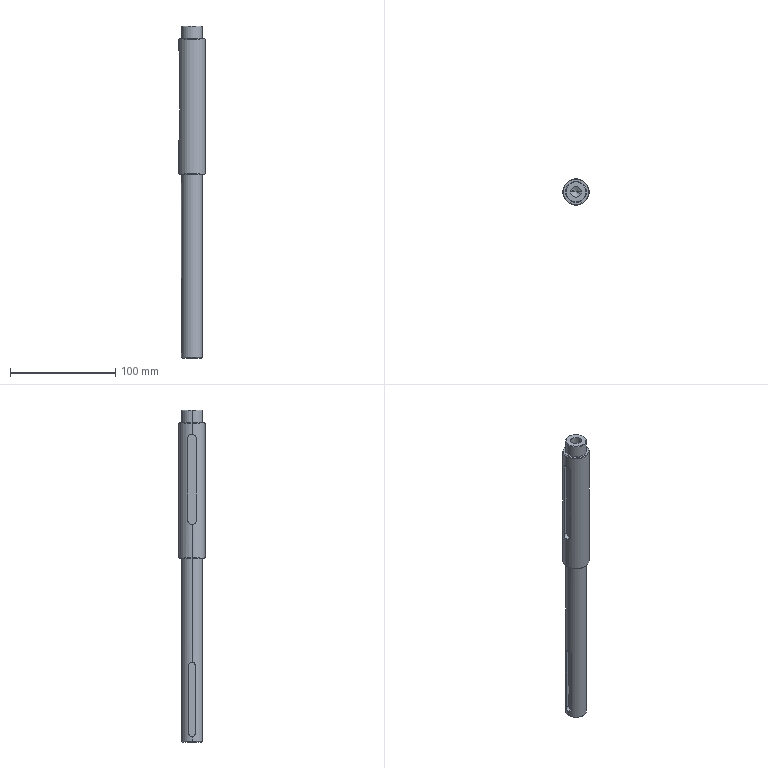Component | SolidWorks | TractionDriveWheelAssembly-1_TractionDriveAxis-1 | 1 solid | 34 faces | box 25 x 25 x 316 mm | volume 116078 mm3 | cylinder 14 | cone 10 | plane 10 | commonest cylinder face diameters 20 x4 6 x3 8 x3 10 x2 25 x2
STEP:
#1=CARTESIAN_POINT('',(-11.988,-1.571,24.075));
#2=VERTEX_POINT('',#1);
#3=CARTESIAN_POINT('',(-11.595,-1.571,24.075));
#4=VERTEX_POINT('',#3);
#5=CARTESIAN_POINT('',(-11.792,-1.571,24.075));
#6=DIRECTION('',(-0.,-0.,1.));
#7=DIRECTION('',(1.,0.,0.));
#8=AXIS2_PLACEMENT_3D('',#5,#6,#7);
#9=CIRCLE('',#8,0.1969);
#10=EDGE_CURVE('',#2,#4,#9,.T.);
#11=ORIENTED_EDGE('',*,*,#10,.F.);
#12=CARTESIAN_POINT('',(-11.988,-1.571,25.039));
#13=VERTEX_POINT('',#12);
#14=CARTESIAN_POINT('',(-11.988,-1.571,25.039));
#15=DIRECTION('',(-0.,-0.,1.));
#16=VECTOR('',#15,39.37);
#17=LINE('',#14,#16);
#18=EDGE_CURVE('',#2,#13,#17,.T.);
#19=ORIENTED_EDGE('',*,*,#18,.T.);
#20=CARTESIAN_POINT('',(-11.595,-1.571,25.039));
#21=VERTEX_POINT('',#20);
#22=CARTESIAN_POINT('',(-11.792,-1.571,25.039));
#23=DIRECTION('',(-0.,-0.,1.));
#24=DIRECTION('',(1.,0.,0.));
#25=AXIS2_PLACEMENT_3D('',#22,#23,#24);
#26=CIRCLE('',#25,0.1969);
#27=EDGE_CURVE('',#13,#21,#26,.T.);
#28=ORIENTED_EDGE('',*,*,#27,.T.);
#29=CARTESIAN_POINT('',(-11.595,-1.571,25.039));
#30=DIRECTION('',(-0.,-0.,1.));
#31=VECTOR('',#30,39.37);
#32=LINE('',#29,#31);
#33=EDGE_CURVE('',#4,#21,#32,.T.);
#34=ORIENTED_EDGE('',*,*,#33,.F.);
#35=EDGE_LOOP('',(#11,#19,#28,#34));
#36=FACE_OUTER_BOUND('',#35,.T.);
#37=CARTESIAN_POINT('',(-11.792,-1.571,25.039));
#38=DIRECTION('',(-0.,-0.,1.));
#39=DIRECTION('',(1.,0.,0.));
#40=AXIS2_PLACEMENT_3D('',#37,#38,#39);
#41=CYLINDRICAL_SURFACE('',#40,0.1969);
#42=ADVANCED_FACE('',(#36),#41,.F.);
#43=CARTESIAN_POINT('',(-11.792,-1.571,23.957));
#44=VERTEX_POINT('',#43);
#45=CARTESIAN_POINT('',(-11.595,-1.571,24.075));
#46=DIRECTION('',(0.8572,0.,0.515));
#47=VECTOR('',#46,39.37);
#48=LINE('',#45,#47);
#49=EDGE_CURVE('',#44,#4,#48,.T.);
#50=ORIENTED_EDGE('',*,*,#49,.F.);
#51=CARTESIAN_POINT('',(-11.988,-1.571,24.075));
#52=DIRECTION('',(-0.8572,-0.,0.515));
#53=VECTOR('',#52,39.37);
#54=LINE('',#51,#53);
#55=EDGE_CURVE('',#44,#2,#54,.T.);
#56=ORIENTED_EDGE('',*,*,#55,.T.);
#57=ORIENTED_EDGE('',*,*,#10,.T.);
#58=EDGE_LOOP('',(#50,#56,#57));
#59=FACE_OUTER_BOUND('',#58,.T.);
#60=CARTESIAN_POINT('',(-11.792,-1.571,24.075));
#61=DIRECTION('',(-0.,-0.,1.));
#62=DIRECTION('',(1.,0.,0.));
#63=AXIS2_PLACEMENT_3D('',#60,#61,#62);
#64=CONICAL_SURFACE('',#63,0.1969,1.03);
#65=ADVANCED_FACE('',(#59),#64,.F.);
#66=CARTESIAN_POINT('',(-12.185,-1.571,12.795));
#67=VERTEX_POINT('',#66);
#68=CARTESIAN_POINT('',(-12.167,-1.453,12.913));
#69=VERTEX_POINT('',#68);
#70=CARTESIAN_POINT('',(-12.185,-1.571,12.795));
#71=CARTESIAN_POINT('',(-12.185,-1.564,12.795));
#72=CARTESIAN_POINT('',(-12.185,-1.556,12.796));
#73=CARTESIAN_POINT('',(-12.184,-1.541,12.799));
#74=CARTESIAN_POINT('',(-12.184,-1.533,12.801));
#75=CARTESIAN_POINT('',(-12.182,-1.519,12.807));
#76=CARTESIAN_POINT('',(-12.181,-1.512,12.811));
#77=CARTESIAN_POINT('',(-12.179,-1.499,12.82));
#78=CARTESIAN_POINT('',(-12.178,-1.493,12.824));
#79=CARTESIAN_POINT('',(-12.175,-1.482,12.835));
#80=CARTESIAN_POINT('',(-12.174,-1.477,12.841));
#81=CARTESIAN_POINT('',(-12.172,-1.469,12.854));
#82=CARTESIAN_POINT('',(-12.171,-1.465,12.861));
#83=CARTESIAN_POINT('',(-12.169,-1.459,12.875));
#84=CARTESIAN_POINT('',(-12.168,-1.457,12.882));
#85=CARTESIAN_POINT('',(-12.167,-1.454,12.898));
#86=CARTESIAN_POINT('',(-12.167,-1.453,12.906));
#87=CARTESIAN_POINT('',(-12.167,-1.453,12.913));
#88=B_SPLINE_CURVE_WITH_KNOTS('',3,(#70,#71,#72,#73,#74,#75,#76,#77,#78,#79,#80,#81,#82,#83,#84,#85,#86,#87),.UNSPECIFIED.,.F.,.F.,(4,2,2,2,2,2,2,2,4),(0.004718,0.005307,0.005896,0.006485,0.007074,0.007663,0.008252,0.008842,0.009431),.UNSPECIFIED.);
#89=EDGE_CURVE('',#67,#69,#88,.T.);
#90=ORIENTED_EDGE('',*,*,#89,.F.);
#91=CARTESIAN_POINT('',(-12.048,-1.571,12.795));
#92=VERTEX_POINT('',#91);
#93=CARTESIAN_POINT('',(-12.284,-1.571,12.795));
#94=DIRECTION('',(1.,0.,0.));
#95=VECTOR('',#94,39.37);
#96=LINE('',#93,#95);
#97=EDGE_CURVE('',#67,#92,#96,.T.);
#98=ORIENTED_EDGE('',*,*,#97,.T.);
#99=CARTESIAN_POINT('',(-12.048,-1.453,12.913));
#100=VERTEX_POINT('',#99);
#101=CARTESIAN_POINT('',(-12.048,-1.571,12.913));
#102=DIRECTION('',(1.,0.,0.));
#103=DIRECTION('',(0.,0.,-1.));
#104=AXIS2_PLACEMENT_3D('',#101,#102,#103);
#105=CIRCLE('',#104,0.1181);
#106=EDGE_CURVE('',#92,#100,#105,.T.);
#107=ORIENTED_EDGE('',*,*,#106,.T.);
#108=CARTESIAN_POINT('',(-12.284,-1.453,12.913));
#109=DIRECTION('',(1.,0.,0.));
#110=VECTOR('',#109,39.37);
#111=LINE('',#108,#110);
#112=EDGE_CURVE('',#69,#100,#111,.T.);
#113=ORIENTED_EDGE('',*,*,#112,.F.);
#114=EDGE_LOOP('',(#90,#98,#107,#113));
#115=FACE_OUTER_BOUND('',#114,.T.);
#116=CARTESIAN_POINT('',(-12.284,-1.571,12.913));
#117=DIRECTION('',(1.,0.,0.));
#118=DIRECTION('',(0.,0.,-1.));
#119=AXIS2_PLACEMENT_3D('',#116,#117,#118);
#120=CYLINDRICAL_SURFACE('',#119,0.1181);
#121=ADVANCED_FACE('',(#115),#120,.F.);
#122=CARTESIAN_POINT('',(-11.398,-1.571,12.618));
#123=VERTEX_POINT('',#122);
#124=CARTESIAN_POINT('',(-12.185,-1.571,12.618));
#125=VERTEX_POINT('',#124);
#126=CARTESIAN_POINT('',(-11.792,-1.571,12.618));
#127=DIRECTION('',(-0.,-0.,1.));
#128=DIRECTION('',(1.,0.,0.));
#129=AXIS2_PLACEMENT_3D('',#126,#127,#128);
#130=CIRCLE('',#129,0.3937);
#131=EDGE_CURVE('',#123,#125,#130,.T.);
#132=ORIENTED_EDGE('',*,*,#131,.T.);
#133=CARTESIAN_POINT('',(-12.185,-1.571,38.002));
#134=DIRECTION('',(-0.,-0.,1.));
#135=VECTOR('',#134,39.37);
#136=LINE('',#133,#135);
#137=EDGE_CURVE('',#125,#67,#136,.T.);
#138=ORIENTED_EDGE('',*,*,#137,.T.);
#139=ORIENTED_EDGE('',*,*,#89,.T.);
#140=CARTESIAN_POINT('',(-12.167,-1.453,15.472));
#141=VERTEX_POINT('',#140);
#142=CARTESIAN_POINT('',(-12.167,-1.453,38.002));
#143=DIRECTION('',(-0.,-0.,1.));
#144=VECTOR('',#143,39.37);
#145=LINE('',#142,#144);
#146=EDGE_CURVE('',#69,#141,#145,.T.);
#147=ORIENTED_EDGE('',*,*,#146,.T.);
#148=CARTESIAN_POINT('',(-12.185,-1.571,15.591));
#149=VERTEX_POINT('',#148);
#150=CARTESIAN_POINT('',(-12.167,-1.453,15.472));
#151=CARTESIAN_POINT('',(-12.167,-1.453,15.48));
#152=CARTESIAN_POINT('',(-12.167,-1.454,15.488));
#153=CARTESIAN_POINT('',(-12.168,-1.457,15.503));
#154=CARTESIAN_POINT('',(-12.169,-1.459,15.511));
#155=CARTESIAN_POINT('',(-12.171,-1.465,15.525));
#156=CARTESIAN_POINT('',(-12.172,-1.469,15.532));
#157=CARTESIAN_POINT('',(-12.174,-1.477,15.545));
#158=CARTESIAN_POINT('',(-12.175,-1.482,15.551));
#159=CARTESIAN_POINT('',(-12.179,-1.499,15.567));
#160=CARTESIAN_POINT('',(-12.181,-1.512,15.576));
#161=CARTESIAN_POINT('',(-12.184,-1.533,15.584));
#162=CARTESIAN_POINT('',(-12.184,-1.541,15.587));
#163=CARTESIAN_POINT('',(-12.185,-1.556,15.59));
#164=CARTESIAN_POINT('',(-12.185,-1.564,15.591));
#165=CARTESIAN_POINT('',(-12.185,-1.571,15.591));
#166=B_SPLINE_CURVE_WITH_KNOTS('',3,(#150,#151,#152,#153,#154,#155,#156,#157,#158,#159,#160,#161,#162,#163,#164,#165),.UNSPECIFIED.,.F.,.F.,(4,2,2,2,2,2,2,4),(0.,0.0005898,0.00118,0.001769,0.002359,0.003539,0.004128,0.004718),.UNSPECIFIED.);
#167=EDGE_CURVE('',#141,#149,#166,.T.);
#168=ORIENTED_EDGE('',*,*,#167,.T.);
#169=CARTESIAN_POINT('',(-12.185,-1.571,19.488));
#170=VERTEX_POINT('',#169);
#171=CARTESIAN_POINT('',(-12.185,-1.571,38.002));
#172=DIRECTION('',(-0.,-0.,1.));
#173=VECTOR('',#172,39.37);
#174=LINE('',#171,#173);
#175=EDGE_CURVE('',#149,#170,#174,.T.);
#176=ORIENTED_EDGE('',*,*,#175,.T.);
#177=CARTESIAN_POINT('',(-11.398,-1.571,19.488));
#178=VERTEX_POINT('',#177);
#179=CARTESIAN_POINT('',(-11.792,-1.571,19.488));
#180=DIRECTION('',(-0.,-0.,1.));
#181=DIRECTION('',(1.,0.,0.));
#182=AXIS2_PLACEMENT_3D('',#179,#180,#181);
#183=CIRCLE('',#182,0.3937);
#184=EDGE_CURVE('',#178,#170,#183,.T.);
#185=ORIENTED_EDGE('',*,*,#184,.F.);
#186=CARTESIAN_POINT('',(-11.398,-1.571,38.002));
#187=DIRECTION('',(-0.,-0.,1.));
#188=VECTOR('',#187,39.37);
#189=LINE('',#186,#188);
#190=EDGE_CURVE('',#123,#178,#189,.T.);
#191=ORIENTED_EDGE('',*,*,#190,.F.);
#192=EDGE_LOOP('',(#132,#138,#139,#147,#168,#176,#185,#191));
#193=FACE_OUTER_BOUND('',#192,.T.);
#194=CARTESIAN_POINT('',(-11.792,-1.571,38.002));
#195=DIRECTION('',(-0.,-0.,1.));
#196=DIRECTION('',(1.,0.,0.));
#197=AXIS2_PLACEMENT_3D('',#194,#195,#196);
#198=CYLINDRICAL_SURFACE('',#197,0.3937);
#199=ADVANCED_FACE('',(#193),#198,.T.);
#200=CARTESIAN_POINT('',(-12.166,-1.571,12.598));
#201=VERTEX_POINT('',#200);
#202=CARTESIAN_POINT('',(-11.418,-1.571,12.598));
#203=VERTEX_POINT('',#202);
#204=CARTESIAN_POINT('',(-11.792,-1.571,12.598));
#205=DIRECTION('',(0.,0.,-1.));
#206=DIRECTION('',(1.,0.,0.));
#207=AXIS2_PLACEMENT_3D('',#204,#205,#206);
#208=CIRCLE('',#207,0.374);
#209=EDGE_CURVE('',#201,#203,#208,.T.);
#210=ORIENTED_EDGE('',*,*,#209,.F.);
#211=CARTESIAN_POINT('',(-12.185,-1.571,12.618));
#212=DIRECTION('',(-0.7071,-0.,0.7071));
#213=VECTOR('',#212,39.37);
#214=LINE('',#211,#213);
#215=EDGE_CURVE('',#201,#125,#214,.T.);
#216=ORIENTED_EDGE('',*,*,#215,.T.);
#217=ORIENTED_EDGE('',*,*,#131,.F.);
#218=CARTESIAN_POINT('',(-11.398,-1.571,12.618));
#219=DIRECTION('',(0.7071,0.,0.7071));
#220=VECTOR('',#219,39.37);
#221=LINE('',#218,#220);
#222=EDGE_CURVE('',#203,#123,#221,.T.);
#223=ORIENTED_EDGE('',*,*,#222,.F.);
#224=EDGE_LOOP('',(#210,#216,#217,#223));
#225=FACE_OUTER_BOUND('',#224,.T.);
#226=CARTESIAN_POINT('',(-11.792,-1.571,12.618));
#227=DIRECTION('',(-0.,-0.,1.));
#228=DIRECTION('',(1.,0.,0.));
#229=AXIS2_PLACEMENT_3D('',#226,#227,#228);
#230=CONICAL_SURFACE('',#229,0.3937,0.7854);
#231=ADVANCED_FACE('',(#225),#230,.T.);
#232=CARTESIAN_POINT('',(-11.319,-1.571,24.567));
#233=VERTEX_POINT('',#232);
#234=CARTESIAN_POINT('',(-12.264,-1.571,24.567));
#235=VERTEX_POINT('',#234);
#236=CARTESIAN_POINT('',(-11.792,-1.571,24.567));
#237=DIRECTION('',(-0.,-0.,1.));
#238=DIRECTION('',(-1.,-0.,0.));
#239=AXIS2_PLACEMENT_3D('',#236,#237,#238);
#240=CIRCLE('',#239,0.4724);
#241=EDGE_CURVE('',#233,#235,#240,.T.);
#242=ORIENTED_EDGE('',*,*,#241,.F.);
#243=CARTESIAN_POINT('',(-11.299,-1.571,24.547));
#244=VERTEX_POINT('',#243);
#245=CARTESIAN_POINT('',(-11.319,-1.571,24.567));
#246=DIRECTION('',(0.7071,0.,-0.7071));
#247=VECTOR('',#246,39.37);
#248=LINE('',#245,#247);
#249=EDGE_CURVE('',#233,#244,#248,.T.);
#250=ORIENTED_EDGE('',*,*,#249,.T.);
#251=CARTESIAN_POINT('',(-12.284,-1.571,24.547));
#252=VERTEX_POINT('',#251);
#253=CARTESIAN_POINT('',(-11.792,-1.571,24.547));
#254=DIRECTION('',(0.,0.,-1.));
#255=DIRECTION('',(-1.,-0.,0.));
#256=AXIS2_PLACEMENT_3D('',#253,#254,#255);
#257=CIRCLE('',#256,0.4921);
#258=EDGE_CURVE('',#252,#244,#257,.T.);
#259=ORIENTED_EDGE('',*,*,#258,.F.);
#260=CARTESIAN_POINT('',(-12.264,-1.571,24.567));
#261=DIRECTION('',(-0.7071,-0.,-0.7071));
#262=VECTOR('',#261,39.37);
#263=LINE('',#260,#262);
#264=EDGE_CURVE('',#235,#252,#263,.T.);
#265=ORIENTED_EDGE('',*,*,#264,.F.);
#266=EDGE_LOOP('',(#242,#250,#259,#265));
#267=FACE_OUTER_BOUND('',#266,.T.);
#268=CARTESIAN_POINT('',(-11.792,-1.571,24.567));
#269=DIRECTION('',(0.,0.,-1.));
#270=DIRECTION('',(-1.,-0.,0.));
#271=AXIS2_PLACEMENT_3D('',#268,#269,#270);
#272=CONICAL_SURFACE('',#271,0.4724,0.7854);
#273=ADVANCED_FACE('',(#267),#272,.T.);
#274=CARTESIAN_POINT('',(-11.398,-1.571,24.567));
#275=VERTEX_POINT('',#274);
#276=CARTESIAN_POINT('',(-12.185,-1.571,24.567));
#277=VERTEX_POINT('',#276);
#278=CARTESIAN_POINT('',(-11.792,-1.571,24.567));
#279=DIRECTION('',(-0.,-0.,1.));
#280=DIRECTION('',(1.,0.,0.));
#281=AXIS2_PLACEMENT_3D('',#278,#279,#280);
#282=CIRCLE('',#281,0.3937);
#283=EDGE_CURVE('',#275,#277,#282,.T.);
#284=ORIENTED_EDGE('',*,*,#283,.T.);
#285=CARTESIAN_POINT('',(-12.185,-1.571,25.02));
#286=VERTEX_POINT('',#285);
#287=CARTESIAN_POINT('',(-12.185,-1.571,38.002));
#288=DIRECTION('',(-0.,-0.,1.));
#289=VECTOR('',#288,39.37);
#290=LINE('',#287,#289);
#291=EDGE_CURVE('',#277,#286,#290,.T.);
#292=ORIENTED_EDGE('',*,*,#291,.T.);
#293=CARTESIAN_POINT('',(-11.398,-1.571,25.02));
#294=VERTEX_POINT('',#293);
#295=CARTESIAN_POINT('',(-11.792,-1.571,25.02));
#296=DIRECTION('',(0.,0.,-1.));
#297=DIRECTION('',(-1.,-0.,0.));
#298=AXIS2_PLACEMENT_3D('',#295,#296,#297);
#299=CIRCLE('',#298,0.3937);
#300=EDGE_CURVE('',#286,#294,#299,.T.);
#301=ORIENTED_EDGE('',*,*,#300,.T.);
#302=CARTESIAN_POINT('',(-11.398,-1.571,38.002));
#303=DIRECTION('',(-0.,-0.,1.));
#304=VECTOR('',#303,39.37);
#305=LINE('',#302,#304);
#306=EDGE_CURVE('',#275,#294,#305,.T.);
#307=ORIENTED_EDGE('',*,*,#306,.F.);
#308=EDGE_LOOP('',(#284,#292,#301,#307));
#309=FACE_OUTER_BOUND('',#308,.T.);
#310=CARTESIAN_POINT('',(-11.792,-1.571,38.002));
#311=DIRECTION('',(-0.,-0.,1.));
#312=DIRECTION('',(1.,0.,0.));
#313=AXIS2_PLACEMENT_3D('',#310,#311,#312);
#314=CYLINDRICAL_SURFACE('',#313,0.3937);
#315=ADVANCED_FACE('',(#309),#314,.T.);
#316=CARTESIAN_POINT('',(-11.418,-1.571,25.039));
#317=VERTEX_POINT('',#316);
#318=CARTESIAN_POINT('',(-12.166,-1.571,25.039));
#319=VERTEX_POINT('',#318);
#320=CARTESIAN_POINT('',(-11.792,-1.571,25.039));
#321=DIRECTION('',(-0.,-0.,1.));
#322=DIRECTION('',(-1.,-0.,0.));
#323=AXIS2_PLACEMENT_3D('',#320,#321,#322);
#324=CIRCLE('',#323,0.374);
#325=EDGE_CURVE('',#317,#319,#324,.T.);
#326=ORIENTED_EDGE('',*,*,#325,.F.);
#327=CARTESIAN_POINT('',(-11.418,-1.571,25.039));
#328=DIRECTION('',(0.7071,0.,-0.7071));
#329=VECTOR('',#328,39.37);
#330=LINE('',#327,#329);
#331=EDGE_CURVE('',#317,#294,#330,.T.);
#332=ORIENTED_EDGE('',*,*,#331,.T.);
#333=ORIENTED_EDGE('',*,*,#300,.F.);
#334=CARTESIAN_POINT('',(-12.166,-1.571,25.039));
#335=DIRECTION('',(-0.7071,-0.,-0.7071));
#336=VECTOR('',#335,39.37);
#337=LINE('',#334,#336);
#338=EDGE_CURVE('',#319,#286,#337,.T.);
#339=ORIENTED_EDGE('',*,*,#338,.F.);
#340=EDGE_LOOP('',(#326,#332,#333,#339));
#341=FACE_OUTER_BOUND('',#340,.T.);
#342=CARTESIAN_POINT('',(-11.792,-1.571,25.039));
#343=DIRECTION('',(0.,0.,-1.));
#344=DIRECTION('',(-1.,-0.,0.));
#345=AXIS2_PLACEMENT_3D('',#342,#343,#344);
#346=CONICAL_SURFACE('',#345,0.374,0.7854);
#347=ADVANCED_FACE('',(#341),#346,.T.);
#348=CARTESIAN_POINT('',(-12.284,-1.571,20.748));
#349=VERTEX_POINT('',#348);
#350=CARTESIAN_POINT('',(-12.258,-1.414,20.906));
#351=VERTEX_POINT('',#350);
#352=CARTESIAN_POINT('',(-12.284,-1.571,20.748));
#353=CARTESIAN_POINT('',(-12.284,-1.561,20.748));
#354=CARTESIAN_POINT('',(-12.283,-1.55,20.749));
#355=CARTESIAN_POINT('',(-12.282,-1.53,20.753));
#356=CARTESIAN_POINT('',(-12.281,-1.52,20.756));
#357=CARTESIAN_POINT('',(-12.279,-1.501,20.764));
#358=CARTESIAN_POINT('',(-12.277,-1.492,20.769));
#359=CARTESIAN_POINT('',(-12.274,-1.475,20.78));
#360=CARTESIAN_POINT('',(-12.273,-1.467,20.787));
#361=CARTESIAN_POINT('',(-12.269,-1.453,20.801));
#362=CARTESIAN_POINT('',(-12.268,-1.446,20.809));
#363=CARTESIAN_POINT('',(-12.264,-1.435,20.826));
#364=CARTESIAN_POINT('',(-12.263,-1.43,20.835));
#365=CARTESIAN_POINT('',(-12.261,-1.422,20.854));
#366=CARTESIAN_POINT('',(-12.26,-1.419,20.864));
#367=CARTESIAN_POINT('',(-12.258,-1.415,20.885));
#368=CARTESIAN_POINT('',(-12.258,-1.414,20.895));
#369=CARTESIAN_POINT('',(-12.258,-1.414,20.906));
#370=B_SPLINE_CURVE_WITH_KNOTS('',3,(#352,#353,#354,#355,#356,#357,#358,#359,#360,#361,#362,#363,#364,#365,#366,#367,#368,#369),.UNSPECIFIED.,.F.,.F.,(4,2,2,2,2,2,2,2,4),(0.006296,0.007082,0.007868,0.008654,0.00944,0.01023,0.01101,0.0118,0.01258),.UNSPECIFIED.);
#371=EDGE_CURVE('',#349,#351,#370,.T.);
#372=ORIENTED_EDGE('',*,*,#371,.F.);
#373=CARTESIAN_POINT('',(-12.126,-1.571,20.748));
#374=VERTEX_POINT('',#373);
#375=CARTESIAN_POINT('',(-12.284,-1.571,20.748));
#376=DIRECTION('',(1.,0.,0.));
#377=VECTOR('',#376,39.37);
#378=LINE('',#375,#377);
#379=EDGE_CURVE('',#349,#374,#378,.T.);
#380=ORIENTED_EDGE('',*,*,#379,.T.);
#381=CARTESIAN_POINT('',(-12.126,-1.414,20.906));
#382=VERTEX_POINT('',#381);
#383=CARTESIAN_POINT('',(-12.126,-1.571,20.906));
#384=DIRECTION('',(1.,0.,0.));
#385=DIRECTION('',(0.,0.,-1.));
#386=AXIS2_PLACEMENT_3D('',#383,#384,#385);
#387=CIRCLE('',#386,0.1575);
#388=EDGE_CURVE('',#374,#382,#387,.T.);
#389=ORIENTED_EDGE('',*,*,#388,.T.);
#390=CARTESIAN_POINT('',(-12.284,-1.414,20.906));
#391=DIRECTION('',(1.,0.,0.));
#392=VECTOR('',#391,39.37);
#393=LINE('',#390,#392);
#394=EDGE_CURVE('',#351,#382,#393,.T.);
#395=ORIENTED_EDGE('',*,*,#394,.F.);
#396=EDGE_LOOP('',(#372,#380,#389,#395));
#397=FACE_OUTER_BOUND('',#396,.T.);
#398=CARTESIAN_POINT('',(-12.284,-1.571,20.906));
#399=DIRECTION('',(1.,0.,0.));
#400=DIRECTION('',(0.,0.,-1.));
#401=AXIS2_PLACEMENT_3D('',#398,#399,#400);
#402=CYLINDRICAL_SURFACE('',#401,0.1575);
#403=ADVANCED_FACE('',(#397),#402,.F.);
#404=CARTESIAN_POINT('',(-12.264,-1.571,19.488));
#405=VERTEX_POINT('',#404);
#406=CARTESIAN_POINT('',(-11.319,-1.571,19.488));
#407=VERTEX_POINT('',#406);
#408=CARTESIAN_POINT('',(-11.792,-1.571,19.488));
#409=DIRECTION('',(0.,0.,-1.));
#410=DIRECTION('',(1.,0.,0.));
#411=AXIS2_PLACEMENT_3D('',#408,#409,#410);
#412=CIRCLE('',#411,0.4724);
#413=EDGE_CURVE('',#405,#407,#412,.T.);
#414=ORIENTED_EDGE('',*,*,#413,.F.);
#415=CARTESIAN_POINT('',(-12.284,-1.571,19.508));
#416=VERTEX_POINT('',#415);
#417=CARTESIAN_POINT('',(-12.284,-1.571,19.508));
#418=DIRECTION('',(-0.7071,-0.,0.7071));
#419=VECTOR('',#418,39.37);
#420=LINE('',#417,#419);
#421=EDGE_CURVE('',#405,#416,#420,.T.);
#422=ORIENTED_EDGE('',*,*,#421,.T.);
#423=CARTESIAN_POINT('',(-11.299,-1.571,19.508));
#424=VERTEX_POINT('',#423);
#425=CARTESIAN_POINT('',(-11.792,-1.571,19.508));
#426=DIRECTION('',(-0.,-0.,1.));
#427=DIRECTION('',(1.,0.,0.));
#428=AXIS2_PLACEMENT_3D('',#425,#426,#427);
#429=CIRCLE('',#428,0.4921);
#430=EDGE_CURVE('',#424,#416,#429,.T.);
#431=ORIENTED_EDGE('',*,*,#430,.F.);
#432=CARTESIAN_POINT('',(-11.299,-1.571,19.508));
#433=DIRECTION('',(0.7071,0.,0.7071));
#434=VECTOR('',#433,39.37);
#435=LINE('',#432,#434);
#436=EDGE_CURVE('',#407,#424,#435,.T.);
#437=ORIENTED_EDGE('',*,*,#436,.F.);
#438=EDGE_LOOP('',(#414,#422,#431,#437));
#439=FACE_OUTER_BOUND('',#438,.T.);
#440=CARTESIAN_POINT('',(-11.792,-1.571,19.508));
#441=DIRECTION('',(-0.,-0.,1.));
#442=DIRECTION('',(1.,0.,0.));
#443=AXIS2_PLACEMENT_3D('',#440,#441,#442);
#444=CONICAL_SURFACE('',#443,0.4921,0.7854);
#445=ADVANCED_FACE('',(#439),#444,.T.);
#446=ORIENTED_EDGE('',*,*,#430,.T.);
#447=CARTESIAN_POINT('',(-12.284,-1.571,38.002));
#448=DIRECTION('',(-0.,-0.,1.));
#449=VECTOR('',#448,39.37);
#450=LINE('',#447,#449);
#451=EDGE_CURVE('',#416,#349,#450,.T.);
#452=ORIENTED_EDGE('',*,*,#451,.T.);
#453=ORIENTED_EDGE('',*,*,#371,.T.);
#454=CARTESIAN_POINT('',(-12.258,-1.414,23.976));
#455=VERTEX_POINT('',#454);
#456=CARTESIAN_POINT('',(-12.258,-1.414,38.002));
#457=DIRECTION('',(-0.,-0.,1.));
#458=VECTOR('',#457,39.37);
#459=LINE('',#456,#458);
#460=EDGE_CURVE('',#351,#455,#459,.T.);
#461=ORIENTED_EDGE('',*,*,#460,.T.);
#462=CARTESIAN_POINT('',(-12.284,-1.571,24.134));
#463=VERTEX_POINT('',#462);
#464=CARTESIAN_POINT('',(-12.258,-1.414,23.976));
#465=CARTESIAN_POINT('',(-12.258,-1.414,23.987));
#466=CARTESIAN_POINT('',(-12.258,-1.415,23.997));
#467=CARTESIAN_POINT('',(-12.26,-1.419,24.017));
#468=CARTESIAN_POINT('',(-12.261,-1.422,24.027));
#469=CARTESIAN_POINT('',(-12.263,-1.43,24.046));
#470=CARTESIAN_POINT('',(-12.264,-1.435,24.055));
#471=CARTESIAN_POINT('',(-12.268,-1.446,24.073));
#472=CARTESIAN_POINT('',(-12.269,-1.453,24.081));
#473=CARTESIAN_POINT('',(-12.273,-1.467,24.095));
#474=CARTESIAN_POINT('',(-12.274,-1.475,24.101));
#475=CARTESIAN_POINT('',(-12.277,-1.492,24.113));
#476=CARTESIAN_POINT('',(-12.279,-1.501,24.118));
#477=CARTESIAN_POINT('',(-12.281,-1.52,24.126));
#478=CARTESIAN_POINT('',(-12.282,-1.53,24.129));
#479=CARTESIAN_POINT('',(-12.283,-1.551,24.133));
#480=CARTESIAN_POINT('',(-12.284,-1.561,24.134));
#481=CARTESIAN_POINT('',(-12.284,-1.571,24.134));
#482=B_SPLINE_CURVE_WITH_KNOTS('',3,(#464,#465,#466,#467,#468,#469,#470,#471,#472,#473,#474,#475,#476,#477,#478,#479,#480,#481),.UNSPECIFIED.,.F.,.F.,(4,2,2,2,2,2,2,2,4),(0.,0.000787,0.001574,0.002361,0.003148,0.003935,0.004722,0.005509,0.006296),.UNSPECIFIED.);
#483=EDGE_CURVE('',#455,#463,#482,.T.);
#484=ORIENTED_EDGE('',*,*,#483,.T.);
#485=CARTESIAN_POINT('',(-12.284,-1.571,38.002));
#486=DIRECTION('',(-0.,-0.,1.));
#487=VECTOR('',#486,39.37);
#488=LINE('',#485,#487);
#489=EDGE_CURVE('',#463,#252,#488,.T.);
#490=ORIENTED_EDGE('',*,*,#489,.T.);
#491=ORIENTED_EDGE('',*,*,#258,.T.);
#492=CARTESIAN_POINT('',(-11.299,-1.571,38.002));
#493=DIRECTION('',(-0.,-0.,1.));
#494=VECTOR('',#493,39.37);
#495=LINE('',#492,#494);
#496=EDGE_CURVE('',#424,#244,#495,.T.);
#497=ORIENTED_EDGE('',*,*,#496,.F.);
#498=EDGE_LOOP('',(#446,#452,#453,#461,#484,#490,#491,#497));
#499=FACE_OUTER_BOUND('',#498,.T.);
#500=CARTESIAN_POINT('',(-11.792,-1.571,38.002));
#501=DIRECTION('',(-0.,-0.,1.));
#502=DIRECTION('',(1.,0.,0.));
#503=AXIS2_PLACEMENT_3D('',#500,#501,#502);
#504=CYLINDRICAL_SURFACE('',#503,0.4921);
#505=ADVANCED_FACE('',(#499),#504,.T.);
#506=ORIENTED_EDGE('',*,*,#451,.F.);
#507=CARTESIAN_POINT('',(-11.792,-1.571,19.508));
#508=DIRECTION('',(-0.,-0.,1.));
#509=DIRECTION('',(1.,0.,0.));
#510=AXIS2_PLACEMENT_3D('',#507,#508,#509);
#511=CIRCLE('',#510,0.4921);
#512=EDGE_CURVE('',#416,#424,#511,.T.);
#513=ORIENTED_EDGE('',*,*,#512,.T.);
#514=ORIENTED_EDGE('',*,*,#496,.T.);
#515=CARTESIAN_POINT('',(-11.792,-1.571,24.547));
#516=DIRECTION('',(0.,0.,-1.));
#517=DIRECTION('',(-1.,-0.,0.));
#518=AXIS2_PLACEMENT_3D('',#515,#516,#517);
#519=CIRCLE('',#518,0.4921);
#520=EDGE_CURVE('',#244,#252,#519,.T.);
#521=ORIENTED_EDGE('',*,*,#520,.T.);
#522=ORIENTED_EDGE('',*,*,#489,.F.);
#523=CARTESIAN_POINT('',(-12.258,-1.729,23.976));
#524=VERTEX_POINT('',#523);
#525=CARTESIAN_POINT('',(-12.284,-1.571,24.134));
#526=CARTESIAN_POINT('',(-12.284,-1.582,24.134));
#527=CARTESIAN_POINT('',(-12.283,-1.592,24.133));
#528=CARTESIAN_POINT('',(-12.282,-1.612,24.129));
#529=CARTESIAN_POINT('',(-12.281,-1.622,24.126));
#530=CARTESIAN_POINT('',(-12.279,-1.641,24.118));
#531=CARTESIAN_POINT('',(-12.277,-1.65,24.113));
#532=CARTESIAN_POINT('',(-12.274,-1.667,24.102));
#533=CARTESIAN_POINT('',(-12.273,-1.675,24.095));
#534=CARTESIAN_POINT('',(-12.269,-1.69,24.08));
#535=CARTESIAN_POINT('',(-12.268,-1.696,24.073));
#536=CARTESIAN_POINT('',(-12.264,-1.708,24.056));
#537=CARTESIAN_POINT('',(-12.263,-1.713,24.046));
#538=CARTESIAN_POINT('',(-12.261,-1.721,24.027));
#539=CARTESIAN_POINT('',(-12.26,-1.724,24.018));
#540=CARTESIAN_POINT('',(-12.258,-1.728,23.997));
#541=CARTESIAN_POINT('',(-12.258,-1.729,23.987));
#542=CARTESIAN_POINT('',(-12.258,-1.729,23.976));
#543=B_SPLINE_CURVE_WITH_KNOTS('',3,(#525,#526,#527,#528,#529,#530,#531,#532,#533,#534,#535,#536,#537,#538,#539,#540,#541,#542),.UNSPECIFIED.,.F.,.F.,(4,2,2,2,2,2,2,2,4),(0.006296,0.007082,0.007868,0.008654,0.00944,0.01023,0.01101,0.0118,0.01258),.UNSPECIFIED.);
#544=EDGE_CURVE('',#463,#524,#543,.T.);
#545=ORIENTED_EDGE('',*,*,#544,.T.);
#546=CARTESIAN_POINT('',(-12.258,-1.729,20.906));
#547=VERTEX_POINT('',#546);
#548=CARTESIAN_POINT('',(-12.258,-1.729,38.002));
#549=DIRECTION('',(0.,0.,-1.));
#550=VECTOR('',#549,39.37);
#551=LINE('',#548,#550);
#552=EDGE_CURVE('',#524,#547,#551,.T.);
#553=ORIENTED_EDGE('',*,*,#552,.T.);
#554=CARTESIAN_POINT('',(-12.258,-1.729,20.906));
#555=CARTESIAN_POINT('',(-12.258,-1.729,20.895));
#556=CARTESIAN_POINT('',(-12.258,-1.728,20.885));
#557=CARTESIAN_POINT('',(-12.26,-1.724,20.865));
#558=CARTESIAN_POINT('',(-12.261,-1.721,20.854));
#559=CARTESIAN_POINT('',(-12.263,-1.713,20.835));
#560=CARTESIAN_POINT('',(-12.264,-1.708,20.826));
#561=CARTESIAN_POINT('',(-12.268,-1.696,20.809));
#562=CARTESIAN_POINT('',(-12.269,-1.69,20.801));
#563=CARTESIAN_POINT('',(-12.273,-1.675,20.787));
#564=CARTESIAN_POINT('',(-12.274,-1.668,20.78));
#565=CARTESIAN_POINT('',(-12.277,-1.65,20.769));
#566=CARTESIAN_POINT('',(-12.279,-1.641,20.764));
#567=CARTESIAN_POINT('',(-12.281,-1.622,20.756));
#568=CARTESIAN_POINT('',(-12.282,-1.612,20.753));
#569=CARTESIAN_POINT('',(-12.283,-1.592,20.749));
#570=CARTESIAN_POINT('',(-12.284,-1.582,20.748));
#571=CARTESIAN_POINT('',(-12.284,-1.571,20.748));
#572=B_SPLINE_CURVE_WITH_KNOTS('',3,(#554,#555,#556,#557,#558,#559,#560,#561,#562,#563,#564,#565,#566,#567,#568,#569,#570,#571),.UNSPECIFIED.,.F.,.F.,(4,2,2,2,2,2,2,2,4),(0.,0.000787,0.001574,0.002361,0.003148,0.003935,0.004722,0.005509,0.006296),.UNSPECIFIED.);
#573=EDGE_CURVE('',#547,#349,#572,.T.);
#574=ORIENTED_EDGE('',*,*,#573,.T.);
#575=EDGE_LOOP('',(#506,#513,#514,#521,#522,#545,#553,#574));
#576=FACE_OUTER_BOUND('',#575,.T.);
#577=CARTESIAN_POINT('',(-11.792,-1.571,38.002));
#578=DIRECTION('',(-0.,-0.,1.));
#579=DIRECTION('',(1.,0.,0.));
#580=AXIS2_PLACEMENT_3D('',#577,#578,#579);
#581=CYLINDRICAL_SURFACE('',#580,0.4921);
#582=ADVANCED_FACE('',(#576),#581,.T.);
#583=CARTESIAN_POINT('',(-11.792,-1.571,19.488));
#584=DIRECTION('',(0.,0.,-1.));
#585=DIRECTION('',(1.,0.,0.));
#586=AXIS2_PLACEMENT_3D('',#583,#584,#585);
#587=CIRCLE('',#586,0.4724);
#588=EDGE_CURVE('',#407,#405,#587,.T.);
#589=ORIENTED_EDGE('',*,*,#588,.T.);
#590=ORIENTED_EDGE('',*,*,#413,.T.);
#591=EDGE_LOOP('',(#589,#590));
#592=FACE_OUTER_BOUND('',#591,.T.);
#593=ORIENTED_EDGE('',*,*,#184,.T.);
#594=CARTESIAN_POINT('',(-11.792,-1.571,19.488));
#595=DIRECTION('',(-0.,-0.,1.));
#596=DIRECTION('',(1.,0.,0.));
#597=AXIS2_PLACEMENT_3D('',#594,#595,#596);
#598=CIRCLE('',#597,0.3937);
#599=EDGE_CURVE('',#170,#178,#598,.T.);
#600=ORIENTED_EDGE('',*,*,#599,.T.);
#601=EDGE_LOOP('',(#593,#600));
#602=FACE_BOUND('',#601,.T.);
#603=CARTESIAN_POINT('',(-11.792,-1.079,19.488));
#604=DIRECTION('',(-0.,-0.,1.));
#605=DIRECTION('',(1.,0.,0.));
#606=AXIS2_PLACEMENT_3D('',#603,#604,#605);
#607=PLANE('',#606);
#608=ADVANCED_FACE('',(#592,#602),#607,.F.);
#609=ORIENTED_EDGE('',*,*,#421,.F.);
#610=ORIENTED_EDGE('',*,*,#588,.F.);
#611=ORIENTED_EDGE('',*,*,#436,.T.);
#612=ORIENTED_EDGE('',*,*,#512,.F.);
#613=EDGE_LOOP('',(#609,#610,#611,#612));
#614=FACE_OUTER_BOUND('',#613,.T.);
#615=CARTESIAN_POINT('',(-11.792,-1.571,19.508));
#616=DIRECTION('',(-0.,-0.,1.));
#617=DIRECTION('',(1.,0.,0.));
#618=AXIS2_PLACEMENT_3D('',#615,#616,#617);
#619=CONICAL_SURFACE('',#618,0.4921,0.7854);
#620=ADVANCED_FACE('',(#614),#619,.T.);
#621=CARTESIAN_POINT('',(-12.126,-1.414,23.976));
#622=VERTEX_POINT('',#621);
#623=CARTESIAN_POINT('',(-12.284,-1.414,23.976));
#624=DIRECTION('',(1.,0.,0.));
#625=VECTOR('',#624,39.37);
#626=LINE('',#623,#625);
#627=EDGE_CURVE('',#455,#622,#626,.T.);
#628=ORIENTED_EDGE('',*,*,#627,.T.);
#629=CARTESIAN_POINT('',(-12.126,-1.729,23.976));
#630=VERTEX_POINT('',#629);
#631=CARTESIAN_POINT('',(-12.126,-1.571,23.976));
#632=DIRECTION('',(1.,0.,0.));
#633=DIRECTION('',(0.,0.,-1.));
#634=AXIS2_PLACEMENT_3D('',#631,#632,#633);
#635=CIRCLE('',#634,0.1575);
#636=EDGE_CURVE('',#622,#630,#635,.T.);
#637=ORIENTED_EDGE('',*,*,#636,.T.);
#638=CARTESIAN_POINT('',(-12.284,-1.729,23.976));
#639=DIRECTION('',(1.,0.,0.));
#640=VECTOR('',#639,39.37);
#641=LINE('',#638,#640);
#642=EDGE_CURVE('',#524,#630,#641,.T.);
#643=ORIENTED_EDGE('',*,*,#642,.F.);
#644=ORIENTED_EDGE('',*,*,#544,.F.);
#645=ORIENTED_EDGE('',*,*,#483,.F.);
#646=EDGE_LOOP('',(#628,#637,#643,#644,#645));
#647=FACE_OUTER_BOUND('',#646,.T.);
#648=CARTESIAN_POINT('',(-12.284,-1.571,23.976));
#649=DIRECTION('',(1.,0.,0.));
#650=DIRECTION('',(0.,0.,-1.));
#651=AXIS2_PLACEMENT_3D('',#648,#649,#650);
#652=CYLINDRICAL_SURFACE('',#651,0.1575);
#653=ADVANCED_FACE('',(#647),#652,.F.);
#654=ORIENTED_EDGE('',*,*,#394,.T.);
#655=CARTESIAN_POINT('',(-12.126,-1.414,23.976));
#656=DIRECTION('',(-0.,-0.,1.));
#657=VECTOR('',#656,39.37);
#658=LINE('',#655,#657);
#659=EDGE_CURVE('',#382,#622,#658,.T.);
#660=ORIENTED_EDGE('',*,*,#659,.T.);
#661=ORIENTED_EDGE('',*,*,#627,.F.);
#662=ORIENTED_EDGE('',*,*,#460,.F.);
#663=EDGE_LOOP('',(#654,#660,#661,#662));
#664=FACE_OUTER_BOUND('',#663,.T.);
#665=CARTESIAN_POINT('',(-12.284,-1.414,23.976));
#666=DIRECTION('',(-0.,1.,0.));
#667=DIRECTION('',(1.,0.,0.));
#668=AXIS2_PLACEMENT_3D('',#665,#666,#667);
#669=PLANE('',#668);
#670=ADVANCED_FACE('',(#664),#669,.F.);
#671=ORIENTED_EDGE('',*,*,#379,.F.);
#672=ORIENTED_EDGE('',*,*,#573,.F.);
#673=CARTESIAN_POINT('',(-12.126,-1.729,20.906));
#674=VERTEX_POINT('',#673);
#675=CARTESIAN_POINT('',(-12.284,-1.729,20.906));
#676=DIRECTION('',(1.,0.,0.));
#677=VECTOR('',#676,39.37);
#678=LINE('',#675,#677);
#679=EDGE_CURVE('',#547,#674,#678,.T.);
#680=ORIENTED_EDGE('',*,*,#679,.T.);
#681=CARTESIAN_POINT('',(-12.126,-1.571,20.906));
#682=DIRECTION('',(1.,0.,0.));
#683=DIRECTION('',(0.,0.,-1.));
#684=AXIS2_PLACEMENT_3D('',#681,#682,#683);
#685=CIRCLE('',#684,0.1575);
#686=EDGE_CURVE('',#674,#374,#685,.T.);
#687=ORIENTED_EDGE('',*,*,#686,.T.);
#688=EDGE_LOOP('',(#671,#672,#680,#687));
#689=FACE_OUTER_BOUND('',#688,.T.);
#690=CARTESIAN_POINT('',(-12.284,-1.571,20.906));
#691=DIRECTION('',(1.,0.,0.));
#692=DIRECTION('',(0.,0.,-1.));
#693=AXIS2_PLACEMENT_3D('',#690,#691,#692);
#694=CYLINDRICAL_SURFACE('',#693,0.1575);
#695=ADVANCED_FACE('',(#689),#694,.F.);
#696=ORIENTED_EDGE('',*,*,#642,.T.);
#697=CARTESIAN_POINT('',(-12.126,-1.729,23.976));
#698=DIRECTION('',(0.,0.,-1.));
#699=VECTOR('',#698,39.37);
#700=LINE('',#697,#699);
#701=EDGE_CURVE('',#630,#674,#700,.T.);
#702=ORIENTED_EDGE('',*,*,#701,.T.);
#703=ORIENTED_EDGE('',*,*,#679,.F.);
#704=ORIENTED_EDGE('',*,*,#552,.F.);
#705=EDGE_LOOP('',(#696,#702,#703,#704));
#706=FACE_OUTER_BOUND('',#705,.T.);
#707=CARTESIAN_POINT('',(-12.284,-1.729,23.976));
#708=DIRECTION('',(0.,-1.,-0.));
#709=DIRECTION('',(-1.,-0.,-0.));
#710=AXIS2_PLACEMENT_3D('',#707,#708,#709);
#711=PLANE('',#710);
#712=ADVANCED_FACE('',(#706),#711,.F.);
#713=ORIENTED_EDGE('',*,*,#636,.F.);
#714=ORIENTED_EDGE('',*,*,#659,.F.);
#715=ORIENTED_EDGE('',*,*,#388,.F.);
#716=ORIENTED_EDGE('',*,*,#686,.F.);
#717=ORIENTED_EDGE('',*,*,#701,.F.);
#718=EDGE_LOOP('',(#713,#714,#715,#716,#717));
#719=FACE_OUTER_BOUND('',#718,.T.);
#720=CARTESIAN_POINT('',(-12.126,-1.571,23.976));
#721=DIRECTION('',(1.,0.,0.));
#722=DIRECTION('',(0.,0.,-1.));
#723=AXIS2_PLACEMENT_3D('',#720,#721,#722);
#724=PLANE('',#723);
#725=ADVANCED_FACE('',(#719),#724,.F.);
#726=CARTESIAN_POINT('',(-11.792,-1.571,25.039));
#727=DIRECTION('',(-0.,-0.,1.));
#728=DIRECTION('',(1.,0.,0.));
#729=AXIS2_PLACEMENT_3D('',#726,#727,#728);
#730=CIRCLE('',#729,0.1969);
#731=EDGE_CURVE('',#21,#13,#730,.T.);
#732=ORIENTED_EDGE('',*,*,#731,.F.);
#733=ORIENTED_EDGE('',*,*,#27,.F.);
#734=EDGE_LOOP('',(#732,#733));
#735=FACE_BOUND('',#734,.T.);
#736=CARTESIAN_POINT('',(-11.792,-1.571,25.039));
#737=DIRECTION('',(-0.,-0.,1.));
#738=DIRECTION('',(-1.,-0.,0.));
#739=AXIS2_PLACEMENT_3D('',#736,#737,#738);
#740=CIRCLE('',#739,0.374);
#741=EDGE_CURVE('',#319,#317,#740,.T.);
#742=ORIENTED_EDGE('',*,*,#741,.T.);
#743=ORIENTED_EDGE('',*,*,#325,.T.);
#744=EDGE_LOOP('',(#742,#743));
#745=FACE_OUTER_BOUND('',#744,.T.);
#746=CARTESIAN_POINT('',(-11.792,-1.571,25.039));
#747=DIRECTION('',(0.,0.,-1.));
#748=DIRECTION('',(-1.,-0.,-0.));
#749=AXIS2_PLACEMENT_3D('',#746,#747,#748);
#750=PLANE('',#749);
#751=ADVANCED_FACE('',(#735,#745),#750,.F.);
#752=ORIENTED_EDGE('',*,*,#331,.F.);
#753=ORIENTED_EDGE('',*,*,#741,.F.);
#754=ORIENTED_EDGE('',*,*,#338,.T.);
#755=CARTESIAN_POINT('',(-11.792,-1.571,25.02));
#756=DIRECTION('',(0.,0.,-1.));
#757=DIRECTION('',(-1.,-0.,0.));
#758=AXIS2_PLACEMENT_3D('',#755,#756,#757);
#759=CIRCLE('',#758,0.3937);
#760=EDGE_CURVE('',#294,#286,#759,.T.);
#761=ORIENTED_EDGE('',*,*,#760,.F.);
#762=EDGE_LOOP('',(#752,#753,#754,#761));
#763=FACE_OUTER_BOUND('',#762,.T.);
#764=CARTESIAN_POINT('',(-11.792,-1.571,25.039));
#765=DIRECTION('',(0.,0.,-1.));
#766=DIRECTION('',(-1.,-0.,0.));
#767=AXIS2_PLACEMENT_3D('',#764,#765,#766);
#768=CONICAL_SURFACE('',#767,0.374,0.7854);
#769=ADVANCED_FACE('',(#763),#768,.T.);
#770=ORIENTED_EDGE('',*,*,#291,.F.);
#771=CARTESIAN_POINT('',(-11.792,-1.571,24.567));
#772=DIRECTION('',(-0.,-0.,1.));
#773=DIRECTION('',(1.,0.,0.));
#774=AXIS2_PLACEMENT_3D('',#771,#772,#773);
#775=CIRCLE('',#774,0.3937);
#776=EDGE_CURVE('',#277,#275,#775,.T.);
#777=ORIENTED_EDGE('',*,*,#776,.T.);
#778=ORIENTED_EDGE('',*,*,#306,.T.);
#779=ORIENTED_EDGE('',*,*,#760,.T.);
#780=EDGE_LOOP('',(#770,#777,#778,#779));
#781=FACE_OUTER_BOUND('',#780,.T.);
#782=CARTESIAN_POINT('',(-11.792,-1.571,38.002));
#783=DIRECTION('',(-0.,-0.,1.));
#784=DIRECTION('',(1.,0.,0.));
#785=AXIS2_PLACEMENT_3D('',#782,#783,#784);
#786=CYLINDRICAL_SURFACE('',#785,0.3937);
#787=ADVANCED_FACE('',(#781),#786,.T.);
#788=CARTESIAN_POINT('',(-11.792,-1.571,24.567));
#789=DIRECTION('',(-0.,-0.,1.));
#790=DIRECTION('',(-1.,-0.,0.));
#791=AXIS2_PLACEMENT_3D('',#788,#789,#790);
#792=CIRCLE('',#791,0.4724);
#793=EDGE_CURVE('',#235,#233,#792,.T.);
#794=ORIENTED_EDGE('',*,*,#793,.T.);
#795=ORIENTED_EDGE('',*,*,#241,.T.);
#796=EDGE_LOOP('',(#794,#795));
#797=FACE_OUTER_BOUND('',#796,.T.);
#798=ORIENTED_EDGE('',*,*,#283,.F.);
#799=ORIENTED_EDGE('',*,*,#776,.F.);
#800=EDGE_LOOP('',(#798,#799));
#801=FACE_BOUND('',#800,.T.);
#802=CARTESIAN_POINT('',(-11.792,-1.178,24.567));
#803=DIRECTION('',(0.,0.,-1.));
#804=DIRECTION('',(-1.,-0.,-0.));
#805=AXIS2_PLACEMENT_3D('',#802,#803,#804);
#806=PLANE('',#805);
#807=ADVANCED_FACE('',(#797,#801),#806,.F.);
#808=ORIENTED_EDGE('',*,*,#249,.F.);
#809=ORIENTED_EDGE('',*,*,#793,.F.);
#810=ORIENTED_EDGE('',*,*,#264,.T.);
#811=ORIENTED_EDGE('',*,*,#520,.F.);
#812=EDGE_LOOP('',(#808,#809,#810,#811));
#813=FACE_OUTER_BOUND('',#812,.T.);
#814=CARTESIAN_POINT('',(-11.792,-1.571,24.567));
#815=DIRECTION('',(0.,0.,-1.));
#816=DIRECTION('',(-1.,-0.,0.));
#817=AXIS2_PLACEMENT_3D('',#814,#815,#816);
#818=CONICAL_SURFACE('',#817,0.4724,0.7854);
#819=ADVANCED_FACE('',(#813),#818,.T.);
#820=CARTESIAN_POINT('',(-11.792,-1.571,12.598));
#821=DIRECTION('',(0.,0.,-1.));
#822=DIRECTION('',(1.,0.,0.));
#823=AXIS2_PLACEMENT_3D('',#820,#821,#822);
#824=CIRCLE('',#823,0.374);
#825=EDGE_CURVE('',#203,#201,#824,.T.);
#826=ORIENTED_EDGE('',*,*,#825,.T.);
#827=ORIENTED_EDGE('',*,*,#209,.T.);
#828=EDGE_LOOP('',(#826,#827));
#829=FACE_OUTER_BOUND('',#828,.T.);
#830=CARTESIAN_POINT('',(-11.792,-1.178,12.598));
#831=DIRECTION('',(-0.,-0.,1.));
#832=DIRECTION('',(1.,0.,0.));
#833=AXIS2_PLACEMENT_3D('',#830,#831,#832);
#834=PLANE('',#833);
#835=ADVANCED_FACE('',(#829),#834,.F.);
#836=ORIENTED_EDGE('',*,*,#215,.F.);
#837=ORIENTED_EDGE('',*,*,#825,.F.);
#838=ORIENTED_EDGE('',*,*,#222,.T.);
#839=CARTESIAN_POINT('',(-11.792,-1.571,12.618));
#840=DIRECTION('',(-0.,-0.,1.));
#841=DIRECTION('',(1.,0.,0.));
#842=AXIS2_PLACEMENT_3D('',#839,#840,#841);
#843=CIRCLE('',#842,0.3937);
#844=EDGE_CURVE('',#125,#123,#843,.T.);
#845=ORIENTED_EDGE('',*,*,#844,.F.);
#846=EDGE_LOOP('',(#836,#837,#838,#845));
#847=FACE_OUTER_BOUND('',#846,.T.);
#848=CARTESIAN_POINT('',(-11.792,-1.571,12.618));
#849=DIRECTION('',(-0.,-0.,1.));
#850=DIRECTION('',(1.,0.,0.));
#851=AXIS2_PLACEMENT_3D('',#848,#849,#850);
#852=CONICAL_SURFACE('',#851,0.3937,0.7854);
#853=ADVANCED_FACE('',(#847),#852,.T.);
#854=ORIENTED_EDGE('',*,*,#137,.F.);
#855=ORIENTED_EDGE('',*,*,#844,.T.);
#856=ORIENTED_EDGE('',*,*,#190,.T.);
#857=ORIENTED_EDGE('',*,*,#599,.F.);
#858=ORIENTED_EDGE('',*,*,#175,.F.);
#859=CARTESIAN_POINT('',(-12.167,-1.689,15.472));
#860=VERTEX_POINT('',#859);
#861=CARTESIAN_POINT('',(-12.185,-1.571,15.591));
#862=CARTESIAN_POINT('',(-12.185,-1.579,15.591));
#863=CARTESIAN_POINT('',(-12.185,-1.587,15.59));
#864=CARTESIAN_POINT('',(-12.184,-1.602,15.587));
#865=CARTESIAN_POINT('',(-12.184,-1.609,15.584));
#866=CARTESIAN_POINT('',(-12.182,-1.624,15.579));
#867=CARTESIAN_POINT('',(-12.181,-1.631,15.575));
#868=CARTESIAN_POINT('',(-12.179,-1.643,15.566));
#869=CARTESIAN_POINT('',(-12.178,-1.649,15.561));
#870=CARTESIAN_POINT('',(-12.175,-1.66,15.55));
#871=CARTESIAN_POINT('',(-12.174,-1.665,15.545));
#872=CARTESIAN_POINT('',(-12.172,-1.674,15.532));
#873=CARTESIAN_POINT('',(-12.171,-1.677,15.525));
#874=CARTESIAN_POINT('',(-12.169,-1.683,15.511));
#875=CARTESIAN_POINT('',(-12.168,-1.686,15.503));
#876=CARTESIAN_POINT('',(-12.167,-1.689,15.488));
#877=CARTESIAN_POINT('',(-12.167,-1.689,15.48));
#878=CARTESIAN_POINT('',(-12.167,-1.689,15.472));
#879=B_SPLINE_CURVE_WITH_KNOTS('',3,(#861,#862,#863,#864,#865,#866,#867,#868,#869,#870,#871,#872,#873,#874,#875,#876,#877,#878),.UNSPECIFIED.,.F.,.F.,(4,2,2,2,2,2,2,2,4),(0.004718,0.005307,0.005896,0.006485,0.007074,0.007663,0.008252,0.008842,0.009431),.UNSPECIFIED.);
#880=EDGE_CURVE('',#149,#860,#879,.T.);
#881=ORIENTED_EDGE('',*,*,#880,.T.);
#882=CARTESIAN_POINT('',(-12.167,-1.689,12.913));
#883=VERTEX_POINT('',#882);
#884=CARTESIAN_POINT('',(-12.167,-1.689,38.002));
#885=DIRECTION('',(0.,0.,-1.));
#886=VECTOR('',#885,39.37);
#887=LINE('',#884,#886);
#888=EDGE_CURVE('',#860,#883,#887,.T.);
#889=ORIENTED_EDGE('',*,*,#888,.T.);
#890=CARTESIAN_POINT('',(-12.167,-1.689,12.913));
#891=CARTESIAN_POINT('',(-12.167,-1.689,12.906));
#892=CARTESIAN_POINT('',(-12.167,-1.689,12.898));
#893=CARTESIAN_POINT('',(-12.168,-1.686,12.883));
#894=CARTESIAN_POINT('',(-12.169,-1.683,12.875));
#895=CARTESIAN_POINT('',(-12.171,-1.677,12.861));
#896=CARTESIAN_POINT('',(-12.172,-1.674,12.854));
#897=CARTESIAN_POINT('',(-12.174,-1.665,12.841));
#898=CARTESIAN_POINT('',(-12.175,-1.66,12.835));
#899=CARTESIAN_POINT('',(-12.179,-1.644,12.819));
#900=CARTESIAN_POINT('',(-12.181,-1.631,12.81));
#901=CARTESIAN_POINT('',(-12.184,-1.61,12.801));
#902=CARTESIAN_POINT('',(-12.184,-1.602,12.799));
#903=CARTESIAN_POINT('',(-12.185,-1.587,12.796));
#904=CARTESIAN_POINT('',(-12.185,-1.579,12.795));
#905=CARTESIAN_POINT('',(-12.185,-1.571,12.795));
#906=B_SPLINE_CURVE_WITH_KNOTS('',3,(#890,#891,#892,#893,#894,#895,#896,#897,#898,#899,#900,#901,#902,#903,#904,#905),.UNSPECIFIED.,.F.,.F.,(4,2,2,2,2,2,2,4),(0.,0.0005898,0.00118,0.001769,0.002359,0.003539,0.004128,0.004718),.UNSPECIFIED.);
#907=EDGE_CURVE('',#883,#67,#906,.T.);
#908=ORIENTED_EDGE('',*,*,#907,.T.);
#909=EDGE_LOOP('',(#854,#855,#856,#857,#858,#881,#889,#908));
#910=FACE_OUTER_BOUND('',#909,.T.);
#911=CARTESIAN_POINT('',(-11.792,-1.571,38.002));
#912=DIRECTION('',(-0.,-0.,1.));
#913=DIRECTION('',(1.,0.,0.));
#914=AXIS2_PLACEMENT_3D('',#911,#912,#913);
#915=CYLINDRICAL_SURFACE('',#914,0.3937);
#916=ADVANCED_FACE('',(#910),#915,.T.);
#917=CARTESIAN_POINT('',(-12.048,-1.453,15.472));
#918=VERTEX_POINT('',#917);
#919=CARTESIAN_POINT('',(-12.284,-1.453,15.472));
#920=DIRECTION('',(1.,0.,0.));
#921=VECTOR('',#920,39.37);
#922=LINE('',#919,#921);
#923=EDGE_CURVE('',#141,#918,#922,.T.);
#924=ORIENTED_EDGE('',*,*,#923,.T.);
#925=CARTESIAN_POINT('',(-12.048,-1.689,15.472));
#926=VERTEX_POINT('',#925);
#927=CARTESIAN_POINT('',(-12.048,-1.571,15.472));
#928=DIRECTION('',(1.,0.,0.));
#929=DIRECTION('',(0.,0.,-1.));
#930=AXIS2_PLACEMENT_3D('',#927,#928,#929);
#931=CIRCLE('',#930,0.1181);
#932=EDGE_CURVE('',#918,#926,#931,.T.);
#933=ORIENTED_EDGE('',*,*,#932,.T.);
#934=CARTESIAN_POINT('',(-12.284,-1.689,15.472));
#935=DIRECTION('',(1.,0.,0.));
#936=VECTOR('',#935,39.37);
#937=LINE('',#934,#936);
#938=EDGE_CURVE('',#860,#926,#937,.T.);
#939=ORIENTED_EDGE('',*,*,#938,.F.);
#940=ORIENTED_EDGE('',*,*,#880,.F.);
#941=ORIENTED_EDGE('',*,*,#167,.F.);
#942=EDGE_LOOP('',(#924,#933,#939,#940,#941));
#943=FACE_OUTER_BOUND('',#942,.T.);
#944=CARTESIAN_POINT('',(-12.284,-1.571,15.472));
#945=DIRECTION('',(1.,0.,0.));
#946=DIRECTION('',(0.,0.,-1.));
#947=AXIS2_PLACEMENT_3D('',#944,#945,#946);
#948=CYLINDRICAL_SURFACE('',#947,0.1181);
#949=ADVANCED_FACE('',(#943),#948,.F.);
#950=ORIENTED_EDGE('',*,*,#112,.T.);
#951=CARTESIAN_POINT('',(-12.048,-1.453,15.472));
#952=DIRECTION('',(-0.,-0.,1.));
#953=VECTOR('',#952,39.37);
#954=LINE('',#951,#953);
#955=EDGE_CURVE('',#100,#918,#954,.T.);
#956=ORIENTED_EDGE('',*,*,#955,.T.);
#957=ORIENTED_EDGE('',*,*,#923,.F.);
#958=ORIENTED_EDGE('',*,*,#146,.F.);
#959=EDGE_LOOP('',(#950,#956,#957,#958));
#960=FACE_OUTER_BOUND('',#959,.T.);
#961=CARTESIAN_POINT('',(-12.284,-1.453,15.472));
#962=DIRECTION('',(-0.,1.,0.));
#963=DIRECTION('',(-0.,-0.,1.));
#964=AXIS2_PLACEMENT_3D('',#961,#962,#963);
#965=PLANE('',#964);
#966=ADVANCED_FACE('',(#960),#965,.F.);
#967=ORIENTED_EDGE('',*,*,#97,.F.);
#968=ORIENTED_EDGE('',*,*,#907,.F.);
#969=CARTESIAN_POINT('',(-12.048,-1.689,12.913));
#970=VERTEX_POINT('',#969);
#971=CARTESIAN_POINT('',(-12.284,-1.689,12.913));
#972=DIRECTION('',(1.,0.,0.));
#973=VECTOR('',#972,39.37);
#974=LINE('',#971,#973);
#975=EDGE_CURVE('',#883,#970,#974,.T.);
#976=ORIENTED_EDGE('',*,*,#975,.T.);
#977=CARTESIAN_POINT('',(-12.048,-1.571,12.913));
#978=DIRECTION('',(1.,0.,0.));
#979=DIRECTION('',(0.,0.,-1.));
#980=AXIS2_PLACEMENT_3D('',#977,#978,#979);
#981=CIRCLE('',#980,0.1181);
#982=EDGE_CURVE('',#970,#92,#981,.T.);
#983=ORIENTED_EDGE('',*,*,#982,.T.);
#984=EDGE_LOOP('',(#967,#968,#976,#983));
#985=FACE_OUTER_BOUND('',#984,.T.);
#986=CARTESIAN_POINT('',(-12.284,-1.571,12.913));
#987=DIRECTION('',(1.,0.,0.));
#988=DIRECTION('',(0.,0.,-1.));
#989=AXIS2_PLACEMENT_3D('',#986,#987,#988);
#990=CYLINDRICAL_SURFACE('',#989,0.1181);
#991=ADVANCED_FACE('',(#985),#990,.F.);
#992=ORIENTED_EDGE('',*,*,#938,.T.);
#993=CARTESIAN_POINT('',(-12.048,-1.689,15.472));
#994=DIRECTION('',(0.,0.,-1.));
#995=VECTOR('',#994,39.37);
#996=LINE('',#993,#995);
#997=EDGE_CURVE('',#926,#970,#996,.T.);
#998=ORIENTED_EDGE('',*,*,#997,.T.);
#999=ORIENTED_EDGE('',*,*,#975,.F.);
#1000=ORIENTED_EDGE('',*,*,#888,.F.);
#1001=EDGE_LOOP('',(#992,#998,#999,#1000));
#1002=FACE_OUTER_BOUND('',#1001,.T.);
#1003=CARTESIAN_POINT('',(-12.284,-1.689,15.472));
#1004=DIRECTION('',(0.,-1.,-0.));
#1005=DIRECTION('',(0.,0.,-1.));
#1006=AXIS2_PLACEMENT_3D('',#1003,#1004,#1005);
#1007=PLANE('',#1006);
#1008=ADVANCED_FACE('',(#1002),#1007,.F.);
#1009=ORIENTED_EDGE('',*,*,#932,.F.);
#1010=ORIENTED_EDGE('',*,*,#955,.F.);
#1011=ORIENTED_EDGE('',*,*,#106,.F.);
#1012=ORIENTED_EDGE('',*,*,#982,.F.);
#1013=ORIENTED_EDGE('',*,*,#997,.F.);
#1014=EDGE_LOOP('',(#1009,#1010,#1011,#1012,#1013));
#1015=FACE_OUTER_BOUND('',#1014,.T.);
#1016=CARTESIAN_POINT('',(-12.048,-1.571,15.472));
#1017=DIRECTION('',(1.,0.,0.));
#1018=DIRECTION('',(0.,0.,-1.));
#1019=AXIS2_PLACEMENT_3D('',#1016,#1017,#1018);
#1020=PLANE('',#1019);
#1021=ADVANCED_FACE('',(#1015),#1020,.F.);
#1022=ORIENTED_EDGE('',*,*,#55,.F.);
#1023=ORIENTED_EDGE('',*,*,#49,.T.);
#1024=CARTESIAN_POINT('',(-11.792,-1.571,24.075));
#1025=DIRECTION('',(-0.,-0.,1.));
#1026=DIRECTION('',(1.,0.,0.));
#1027=AXIS2_PLACEMENT_3D('',#1024,#1025,#1026);
#1028=CIRCLE('',#1027,0.1969);
#1029=EDGE_CURVE('',#4,#2,#1028,.T.);
#1030=ORIENTED_EDGE('',*,*,#1029,.T.);
#1031=EDGE_LOOP('',(#1022,#1023,#1030));
#1032=FACE_OUTER_BOUND('',#1031,.T.);
#1033=CARTESIAN_POINT('',(-11.792,-1.571,24.075));
#1034=DIRECTION('',(-0.,-0.,1.));
#1035=DIRECTION('',(1.,0.,0.));
#1036=AXIS2_PLACEMENT_3D('',#1033,#1034,#1035);
#1037=CONICAL_SURFACE('',#1036,0.1969,1.03);
#1038=ADVANCED_FACE('',(#1032),#1037,.F.);
#1039=ORIENTED_EDGE('',*,*,#18,.F.);
#1040=ORIENTED_EDGE('',*,*,#1029,.F.);
#1041=ORIENTED_EDGE('',*,*,#33,.T.);
#1042=ORIENTED_EDGE('',*,*,#731,.T.);
#1043=EDGE_LOOP('',(#1039,#1040,#1041,#1042));
#1044=FACE_OUTER_BOUND('',#1043,.T.);
#1045=CARTESIAN_POINT('',(-11.792,-1.571,25.039));
#1046=DIRECTION('',(-0.,-0.,1.));
#1047=DIRECTION('',(1.,0.,0.));
#1048=AXIS2_PLACEMENT_3D('',#1045,#1046,#1047);
#1049=CYLINDRICAL_SURFACE('',#1048,0.1969);
#1050=ADVANCED_FACE('',(#1044),#1049,.F.);
#1051=CLOSED_SHELL('',(#42,#65,#121,#199,#231,#273,#315,#347,#403,#445,#505,#582,#608,#620,#653,#670,#695,#712,#725,#751,#769,#787,#807,#819,#835,#853,#916,#949,#966,#991,#1008,#1021,#1038,#1050));
#1052=MANIFOLD_SOLID_BREP('',#1051);
#1053=CARTESIAN_POINT('',(0.,0.,0.));
#1054=DIRECTION('',(0.,0.,1.));
#1055=DIRECTION('',(1.,0.,0.));
#1056=AXIS2_PLACEMENT_3D('',#1053,#1054,#1055);
#1057=(LENGTH_UNIT()NAMED_UNIT(*)SI_UNIT($,.METRE.));
#1058=LENGTH_MEASURE_WITH_UNIT(LENGTH_MEASURE(0.0254),#1057);
#1059=DIMENSIONAL_EXPONENTS(1.,0.,0.,0.,0.,0.,0.);
#1060=(CONVERSION_BASED_UNIT('',#1058)LENGTH_UNIT()NAMED_UNIT(#1059));
#1061=UNCERTAINTY_MEASURE_WITH_UNIT(LENGTH_MEASURE(0.00001),#1060,'','');
#1062=(NAMED_UNIT(*)PLANE_ANGLE_UNIT()SI_UNIT($,.RADIAN.));
#1063=(NAMED_UNIT(*)SI_UNIT($,.STERADIAN.)SOLID_ANGLE_UNIT());
#1064=(GEOMETRIC_REPRESENTATION_CONTEXT(3)GLOBAL_UNCERTAINTY_ASSIGNED_CONTEXT((#1061))GLOBAL_UNIT_ASSIGNED_CONTEXT((#1060,#1062,#1063))REPRESENTATION_CONTEXT('',''));
#1065=ADVANCED_BREP_SHAPE_REPRESENTATION('',(#1052,#1056),#1064);
#1066=COLOUR_RGB('',0.7922,0.8196,0.9333);
#1067=FILL_AREA_STYLE_COLOUR('',#1066);
#1068=FILL_AREA_STYLE('',(#1067));
#1069=SURFACE_STYLE_FILL_AREA(#1068);
#1070=SURFACE_SIDE_STYLE('',(#1069));
#1071=SURFACE_STYLE_USAGE(.BOTH.,#1070);
#1072=PRESENTATION_STYLE_ASSIGNMENT((#1071));
#1073=STYLED_ITEM('',(#1072),#1052);
#1074=PRESENTATION_LAYER_ASSIGNMENT('','',(#1073));
#1075=(LENGTH_UNIT()NAMED_UNIT(*)SI_UNIT($,.METRE.));
#1076=LENGTH_MEASURE_WITH_UNIT(LENGTH_MEASURE(0.0254),#1075);
#1077=DIMENSIONAL_EXPONENTS(1.,0.,0.,0.,0.,0.,0.);
#1078=(CONVERSION_BASED_UNIT('',#1076)LENGTH_UNIT()NAMED_UNIT(#1077));
#1079=UNCERTAINTY_MEASURE_WITH_UNIT(LENGTH_MEASURE(0.00001),#1078,'','');
#1080=(NAMED_UNIT(*)PLANE_ANGLE_UNIT()SI_UNIT($,.RADIAN.));
#1081=(NAMED_UNIT(*)SI_UNIT($,.STERADIAN.)SOLID_ANGLE_UNIT());
#1082=(GEOMETRIC_REPRESENTATION_CONTEXT(3)GLOBAL_UNCERTAINTY_ASSIGNED_CONTEXT((#1079))GLOBAL_UNIT_ASSIGNED_CONTEXT((#1078,#1080,#1081))REPRESENTATION_CONTEXT('',''));
#1083=MECHANICAL_DESIGN_GEOMETRIC_PRESENTATION_REPRESENTATION('',(#1073),#1082);